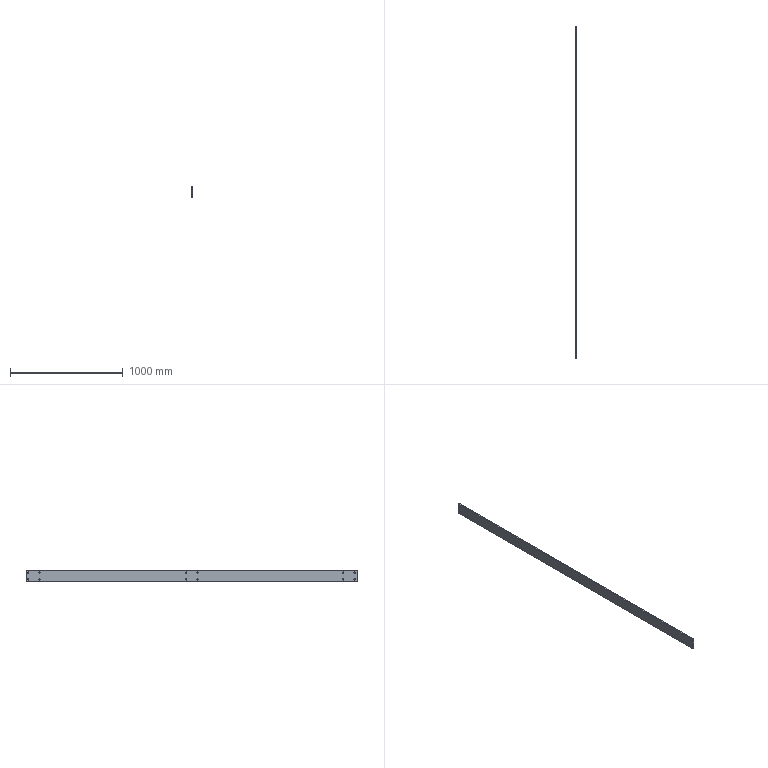Component | SolidWorks | Kick2-2 | 1 solid | 30 faces | box 10 x 2943.5 x 100 mm | volume 2932096 mm3 | cylinder 24 | plane 6 | commonest cylinder face diameters 11 x24 | material Plain Carbon Steel
STEP:
#1=COLOUR_RGB('',0.7922,0.8196,0.9333);
#2=FILL_AREA_STYLE_COLOUR('',#1);
#3=FILL_AREA_STYLE('',(#2));
#4=SURFACE_STYLE_FILL_AREA(#3);
#5=SURFACE_SIDE_STYLE('',(#4));
#6=SURFACE_STYLE_USAGE(.BOTH.,#5);
#7=PRESENTATION_STYLE_ASSIGNMENT((#6));
#8=CARTESIAN_POINT('',(-133.157,36.017,220.491));
#9=VERTEX_POINT('',#8);
#10=CARTESIAN_POINT('',(-133.157,36.017,220.924));
#11=VERTEX_POINT('',#10);
#12=CARTESIAN_POINT('',(-133.157,36.017,220.708));
#13=DIRECTION('',(-1.,0.,-0.));
#14=DIRECTION('',(0.,0.,-1.));
#15=AXIS2_PLACEMENT_3D('',#12,#13,#14);
#16=CIRCLE('',#15,0.2165);
#17=EDGE_CURVE('',#9,#11,#16,.T.);
#18=ORIENTED_EDGE('',*,*,#17,.T.);
#19=CARTESIAN_POINT('',(-132.764,36.017,220.924));
#20=VERTEX_POINT('',#19);
#21=CARTESIAN_POINT('',(-133.157,36.017,220.924));
#22=DIRECTION('',(1.,-0.,0.));
#23=VECTOR('',#22,39.37);
#24=LINE('',#21,#23);
#25=EDGE_CURVE('',#11,#20,#24,.T.);
#26=ORIENTED_EDGE('',*,*,#25,.T.);
#27=CARTESIAN_POINT('',(-132.764,36.017,220.491));
#28=VERTEX_POINT('',#27);
#29=CARTESIAN_POINT('',(-132.764,36.017,220.708));
#30=DIRECTION('',(1.,-0.,0.));
#31=DIRECTION('',(0.,0.,-1.));
#32=AXIS2_PLACEMENT_3D('',#29,#30,#31);
#33=CIRCLE('',#32,0.2165);
#34=EDGE_CURVE('',#20,#28,#33,.T.);
#35=ORIENTED_EDGE('',*,*,#34,.T.);
#36=CARTESIAN_POINT('',(-133.157,36.017,220.491));
#37=DIRECTION('',(1.,-0.,0.));
#38=VECTOR('',#37,39.37);
#39=LINE('',#36,#38);
#40=EDGE_CURVE('',#9,#28,#39,.T.);
#41=ORIENTED_EDGE('',*,*,#40,.F.);
#42=EDGE_LOOP('',(#18,#26,#35,#41));
#43=FACE_OUTER_BOUND('',#42,.T.);
#44=CARTESIAN_POINT('',(-133.157,36.017,220.708));
#45=DIRECTION('',(1.,-0.,0.));
#46=DIRECTION('',(0.,0.,-1.));
#47=AXIS2_PLACEMENT_3D('',#44,#45,#46);
#48=CYLINDRICAL_SURFACE('',#47,0.2165);
#49=ADVANCED_FACE('',(#43),#48,.F.);
#50=CARTESIAN_POINT('',(-133.157,32.08,220.491));
#51=VERTEX_POINT('',#50);
#52=CARTESIAN_POINT('',(-133.157,32.08,220.924));
#53=VERTEX_POINT('',#52);
#54=CARTESIAN_POINT('',(-133.157,32.08,220.708));
#55=DIRECTION('',(-1.,0.,-0.));
#56=DIRECTION('',(0.,0.,-1.));
#57=AXIS2_PLACEMENT_3D('',#54,#55,#56);
#58=CIRCLE('',#57,0.2165);
#59=EDGE_CURVE('',#51,#53,#58,.T.);
#60=ORIENTED_EDGE('',*,*,#59,.T.);
#61=CARTESIAN_POINT('',(-132.764,32.08,220.924));
#62=VERTEX_POINT('',#61);
#63=CARTESIAN_POINT('',(-133.157,32.08,220.924));
#64=DIRECTION('',(1.,-0.,0.));
#65=VECTOR('',#64,39.37);
#66=LINE('',#63,#65);
#67=EDGE_CURVE('',#53,#62,#66,.T.);
#68=ORIENTED_EDGE('',*,*,#67,.T.);
#69=CARTESIAN_POINT('',(-132.764,32.08,220.491));
#70=VERTEX_POINT('',#69);
#71=CARTESIAN_POINT('',(-132.764,32.08,220.708));
#72=DIRECTION('',(1.,-0.,0.));
#73=DIRECTION('',(0.,0.,-1.));
#74=AXIS2_PLACEMENT_3D('',#71,#72,#73);
#75=CIRCLE('',#74,0.2165);
#76=EDGE_CURVE('',#62,#70,#75,.T.);
#77=ORIENTED_EDGE('',*,*,#76,.T.);
#78=CARTESIAN_POINT('',(-133.157,32.08,220.491));
#79=DIRECTION('',(1.,-0.,0.));
#80=VECTOR('',#79,39.37);
#81=LINE('',#78,#80);
#82=EDGE_CURVE('',#51,#70,#81,.T.);
#83=ORIENTED_EDGE('',*,*,#82,.F.);
#84=EDGE_LOOP('',(#60,#68,#77,#83));
#85=FACE_OUTER_BOUND('',#84,.T.);
#86=CARTESIAN_POINT('',(-133.157,32.08,220.708));
#87=DIRECTION('',(1.,-0.,0.));
#88=DIRECTION('',(0.,0.,-1.));
#89=AXIS2_PLACEMENT_3D('',#86,#87,#88);
#90=CYLINDRICAL_SURFACE('',#89,0.2165);
#91=ADVANCED_FACE('',(#85),#90,.F.);
#92=CARTESIAN_POINT('',(-133.157,32.08,222.853));
#93=VERTEX_POINT('',#92);
#94=CARTESIAN_POINT('',(-133.157,32.08,223.286));
#95=VERTEX_POINT('',#94);
#96=CARTESIAN_POINT('',(-133.157,32.08,223.07));
#97=DIRECTION('',(-1.,0.,-0.));
#98=DIRECTION('',(0.,0.,-1.));
#99=AXIS2_PLACEMENT_3D('',#96,#97,#98);
#100=CIRCLE('',#99,0.2165);
#101=EDGE_CURVE('',#93,#95,#100,.T.);
#102=ORIENTED_EDGE('',*,*,#101,.T.);
#103=CARTESIAN_POINT('',(-132.764,32.08,223.286));
#104=VERTEX_POINT('',#103);
#105=CARTESIAN_POINT('',(-133.157,32.08,223.286));
#106=DIRECTION('',(1.,-0.,0.));
#107=VECTOR('',#106,39.37);
#108=LINE('',#105,#107);
#109=EDGE_CURVE('',#95,#104,#108,.T.);
#110=ORIENTED_EDGE('',*,*,#109,.T.);
#111=CARTESIAN_POINT('',(-132.764,32.08,222.853));
#112=VERTEX_POINT('',#111);
#113=CARTESIAN_POINT('',(-132.764,32.08,223.07));
#114=DIRECTION('',(1.,-0.,0.));
#115=DIRECTION('',(0.,0.,-1.));
#116=AXIS2_PLACEMENT_3D('',#113,#114,#115);
#117=CIRCLE('',#116,0.2165);
#118=EDGE_CURVE('',#104,#112,#117,.T.);
#119=ORIENTED_EDGE('',*,*,#118,.T.);
#120=CARTESIAN_POINT('',(-133.157,32.08,222.853));
#121=DIRECTION('',(1.,-0.,0.));
#122=VECTOR('',#121,39.37);
#123=LINE('',#120,#122);
#124=EDGE_CURVE('',#93,#112,#123,.T.);
#125=ORIENTED_EDGE('',*,*,#124,.F.);
#126=EDGE_LOOP('',(#102,#110,#119,#125));
#127=FACE_OUTER_BOUND('',#126,.T.);
#128=CARTESIAN_POINT('',(-133.157,32.08,223.07));
#129=DIRECTION('',(1.,-0.,0.));
#130=DIRECTION('',(0.,0.,-1.));
#131=AXIS2_PLACEMENT_3D('',#128,#129,#130);
#132=CYLINDRICAL_SURFACE('',#131,0.2165);
#133=ADVANCED_FACE('',(#127),#132,.F.);
#134=CARTESIAN_POINT('',(-133.157,-18.846,220.491));
#135=VERTEX_POINT('',#134);
#136=CARTESIAN_POINT('',(-133.157,-18.846,220.924));
#137=VERTEX_POINT('',#136);
#138=CARTESIAN_POINT('',(-133.157,-18.846,220.708));
#139=DIRECTION('',(-1.,0.,-0.));
#140=DIRECTION('',(0.,0.,-1.));
#141=AXIS2_PLACEMENT_3D('',#138,#139,#140);
#142=CIRCLE('',#141,0.2165);
#143=EDGE_CURVE('',#135,#137,#142,.T.);
#144=ORIENTED_EDGE('',*,*,#143,.T.);
#145=CARTESIAN_POINT('',(-132.764,-18.846,220.924));
#146=VERTEX_POINT('',#145);
#147=CARTESIAN_POINT('',(-133.157,-18.846,220.924));
#148=DIRECTION('',(1.,-0.,0.));
#149=VECTOR('',#148,39.37);
#150=LINE('',#147,#149);
#151=EDGE_CURVE('',#137,#146,#150,.T.);
#152=ORIENTED_EDGE('',*,*,#151,.T.);
#153=CARTESIAN_POINT('',(-132.764,-18.846,220.491));
#154=VERTEX_POINT('',#153);
#155=CARTESIAN_POINT('',(-132.764,-18.846,220.708));
#156=DIRECTION('',(1.,-0.,0.));
#157=DIRECTION('',(0.,0.,-1.));
#158=AXIS2_PLACEMENT_3D('',#155,#156,#157);
#159=CIRCLE('',#158,0.2165);
#160=EDGE_CURVE('',#146,#154,#159,.T.);
#161=ORIENTED_EDGE('',*,*,#160,.T.);
#162=CARTESIAN_POINT('',(-133.157,-18.846,220.491));
#163=DIRECTION('',(1.,-0.,0.));
#164=VECTOR('',#163,39.37);
#165=LINE('',#162,#164);
#166=EDGE_CURVE('',#135,#154,#165,.T.);
#167=ORIENTED_EDGE('',*,*,#166,.F.);
#168=EDGE_LOOP('',(#144,#152,#161,#167));
#169=FACE_OUTER_BOUND('',#168,.T.);
#170=CARTESIAN_POINT('',(-133.157,-18.846,220.708));
#171=DIRECTION('',(1.,-0.,0.));
#172=DIRECTION('',(0.,0.,-1.));
#173=AXIS2_PLACEMENT_3D('',#170,#171,#172);
#174=CYLINDRICAL_SURFACE('',#173,0.2165);
#175=ADVANCED_FACE('',(#169),#174,.F.);
#176=CARTESIAN_POINT('',(-133.157,91.135,222.853));
#177=VERTEX_POINT('',#176);
#178=CARTESIAN_POINT('',(-133.157,91.135,223.286));
#179=VERTEX_POINT('',#178);
#180=CARTESIAN_POINT('',(-133.157,91.135,223.07));
#181=DIRECTION('',(-1.,0.,-0.));
#182=DIRECTION('',(0.,0.,-1.));
#183=AXIS2_PLACEMENT_3D('',#180,#181,#182);
#184=CIRCLE('',#183,0.2165);
#185=EDGE_CURVE('',#177,#179,#184,.T.);
#186=ORIENTED_EDGE('',*,*,#185,.T.);
#187=CARTESIAN_POINT('',(-132.764,91.135,223.286));
#188=VERTEX_POINT('',#187);
#189=CARTESIAN_POINT('',(-133.157,91.135,223.286));
#190=DIRECTION('',(1.,-0.,0.));
#191=VECTOR('',#190,39.37);
#192=LINE('',#189,#191);
#193=EDGE_CURVE('',#179,#188,#192,.T.);
#194=ORIENTED_EDGE('',*,*,#193,.T.);
#195=CARTESIAN_POINT('',(-132.764,91.135,222.853));
#196=VERTEX_POINT('',#195);
#197=CARTESIAN_POINT('',(-132.764,91.135,223.07));
#198=DIRECTION('',(1.,-0.,0.));
#199=DIRECTION('',(0.,0.,-1.));
#200=AXIS2_PLACEMENT_3D('',#197,#198,#199);
#201=CIRCLE('',#200,0.2165);
#202=EDGE_CURVE('',#188,#196,#201,.T.);
#203=ORIENTED_EDGE('',*,*,#202,.T.);
#204=CARTESIAN_POINT('',(-133.157,91.135,222.853));
#205=DIRECTION('',(1.,-0.,0.));
#206=VECTOR('',#205,39.37);
#207=LINE('',#204,#206);
#208=EDGE_CURVE('',#177,#196,#207,.T.);
#209=ORIENTED_EDGE('',*,*,#208,.F.);
#210=EDGE_LOOP('',(#186,#194,#203,#209));
#211=FACE_OUTER_BOUND('',#210,.T.);
#212=CARTESIAN_POINT('',(-133.157,91.135,223.07));
#213=DIRECTION('',(1.,-0.,0.));
#214=DIRECTION('',(0.,0.,-1.));
#215=AXIS2_PLACEMENT_3D('',#212,#213,#214);
#216=CYLINDRICAL_SURFACE('',#215,0.2165);
#217=ADVANCED_FACE('',(#211),#216,.F.);
#218=CARTESIAN_POINT('',(-133.157,87.198,220.491));
#219=VERTEX_POINT('',#218);
#220=CARTESIAN_POINT('',(-133.157,87.198,220.924));
#221=VERTEX_POINT('',#220);
#222=CARTESIAN_POINT('',(-133.157,87.198,220.708));
#223=DIRECTION('',(-1.,0.,-0.));
#224=DIRECTION('',(0.,0.,-1.));
#225=AXIS2_PLACEMENT_3D('',#222,#223,#224);
#226=CIRCLE('',#225,0.2165);
#227=EDGE_CURVE('',#219,#221,#226,.T.);
#228=ORIENTED_EDGE('',*,*,#227,.T.);
#229=CARTESIAN_POINT('',(-132.764,87.198,220.924));
#230=VERTEX_POINT('',#229);
#231=CARTESIAN_POINT('',(-133.157,87.198,220.924));
#232=DIRECTION('',(1.,-0.,0.));
#233=VECTOR('',#232,39.37);
#234=LINE('',#231,#233);
#235=EDGE_CURVE('',#221,#230,#234,.T.);
#236=ORIENTED_EDGE('',*,*,#235,.T.);
#237=CARTESIAN_POINT('',(-132.764,87.198,220.491));
#238=VERTEX_POINT('',#237);
#239=CARTESIAN_POINT('',(-132.764,87.198,220.708));
#240=DIRECTION('',(1.,-0.,0.));
#241=DIRECTION('',(0.,0.,-1.));
#242=AXIS2_PLACEMENT_3D('',#239,#240,#241);
#243=CIRCLE('',#242,0.2165);
#244=EDGE_CURVE('',#230,#238,#243,.T.);
#245=ORIENTED_EDGE('',*,*,#244,.T.);
#246=CARTESIAN_POINT('',(-133.157,87.198,220.491));
#247=DIRECTION('',(1.,-0.,0.));
#248=VECTOR('',#247,39.37);
#249=LINE('',#246,#248);
#250=EDGE_CURVE('',#219,#238,#249,.T.);
#251=ORIENTED_EDGE('',*,*,#250,.F.);
#252=EDGE_LOOP('',(#228,#236,#245,#251));
#253=FACE_OUTER_BOUND('',#252,.T.);
#254=CARTESIAN_POINT('',(-133.157,87.198,220.708));
#255=DIRECTION('',(1.,-0.,0.));
#256=DIRECTION('',(0.,0.,-1.));
#257=AXIS2_PLACEMENT_3D('',#254,#255,#256);
#258=CYLINDRICAL_SURFACE('',#257,0.2165);
#259=ADVANCED_FACE('',(#253),#258,.F.);
#260=CARTESIAN_POINT('',(-133.157,87.198,222.853));
#261=VERTEX_POINT('',#260);
#262=CARTESIAN_POINT('',(-133.157,87.198,223.286));
#263=VERTEX_POINT('',#262);
#264=CARTESIAN_POINT('',(-133.157,87.198,223.07));
#265=DIRECTION('',(-1.,0.,-0.));
#266=DIRECTION('',(0.,0.,-1.));
#267=AXIS2_PLACEMENT_3D('',#264,#265,#266);
#268=CIRCLE('',#267,0.2165);
#269=EDGE_CURVE('',#261,#263,#268,.T.);
#270=ORIENTED_EDGE('',*,*,#269,.T.);
#271=CARTESIAN_POINT('',(-132.764,87.198,223.286));
#272=VERTEX_POINT('',#271);
#273=CARTESIAN_POINT('',(-133.157,87.198,223.286));
#274=DIRECTION('',(1.,-0.,0.));
#275=VECTOR('',#274,39.37);
#276=LINE('',#273,#275);
#277=EDGE_CURVE('',#263,#272,#276,.T.);
#278=ORIENTED_EDGE('',*,*,#277,.T.);
#279=CARTESIAN_POINT('',(-132.764,87.198,222.853));
#280=VERTEX_POINT('',#279);
#281=CARTESIAN_POINT('',(-132.764,87.198,223.07));
#282=DIRECTION('',(1.,-0.,0.));
#283=DIRECTION('',(0.,0.,-1.));
#284=AXIS2_PLACEMENT_3D('',#281,#282,#283);
#285=CIRCLE('',#284,0.2165);
#286=EDGE_CURVE('',#272,#280,#285,.T.);
#287=ORIENTED_EDGE('',*,*,#286,.T.);
#288=CARTESIAN_POINT('',(-133.157,87.198,222.853));
#289=DIRECTION('',(1.,-0.,0.));
#290=VECTOR('',#289,39.37);
#291=LINE('',#288,#290);
#292=EDGE_CURVE('',#261,#280,#291,.T.);
#293=ORIENTED_EDGE('',*,*,#292,.F.);
#294=EDGE_LOOP('',(#270,#278,#287,#293));
#295=FACE_OUTER_BOUND('',#294,.T.);
#296=CARTESIAN_POINT('',(-133.157,87.198,223.07));
#297=DIRECTION('',(1.,-0.,0.));
#298=DIRECTION('',(0.,0.,-1.));
#299=AXIS2_PLACEMENT_3D('',#296,#297,#298);
#300=CYLINDRICAL_SURFACE('',#299,0.2165);
#301=ADVANCED_FACE('',(#295),#300,.F.);
#302=CARTESIAN_POINT('',(-133.157,36.017,222.853));
#303=VERTEX_POINT('',#302);
#304=CARTESIAN_POINT('',(-133.157,36.017,223.286));
#305=VERTEX_POINT('',#304);
#306=CARTESIAN_POINT('',(-133.157,36.017,223.07));
#307=DIRECTION('',(-1.,0.,-0.));
#308=DIRECTION('',(0.,0.,-1.));
#309=AXIS2_PLACEMENT_3D('',#306,#307,#308);
#310=CIRCLE('',#309,0.2165);
#311=EDGE_CURVE('',#303,#305,#310,.T.);
#312=ORIENTED_EDGE('',*,*,#311,.T.);
#313=CARTESIAN_POINT('',(-132.764,36.017,223.286));
#314=VERTEX_POINT('',#313);
#315=CARTESIAN_POINT('',(-133.157,36.017,223.286));
#316=DIRECTION('',(1.,-0.,0.));
#317=VECTOR('',#316,39.37);
#318=LINE('',#315,#317);
#319=EDGE_CURVE('',#305,#314,#318,.T.);
#320=ORIENTED_EDGE('',*,*,#319,.T.);
#321=CARTESIAN_POINT('',(-132.764,36.017,222.853));
#322=VERTEX_POINT('',#321);
#323=CARTESIAN_POINT('',(-132.764,36.017,223.07));
#324=DIRECTION('',(1.,-0.,0.));
#325=DIRECTION('',(0.,0.,-1.));
#326=AXIS2_PLACEMENT_3D('',#323,#324,#325);
#327=CIRCLE('',#326,0.2165);
#328=EDGE_CURVE('',#314,#322,#327,.T.);
#329=ORIENTED_EDGE('',*,*,#328,.T.);
#330=CARTESIAN_POINT('',(-133.157,36.017,222.853));
#331=DIRECTION('',(1.,-0.,0.));
#332=VECTOR('',#331,39.37);
#333=LINE('',#330,#332);
#334=EDGE_CURVE('',#303,#322,#333,.T.);
#335=ORIENTED_EDGE('',*,*,#334,.F.);
#336=EDGE_LOOP('',(#312,#320,#329,#335));
#337=FACE_OUTER_BOUND('',#336,.T.);
#338=CARTESIAN_POINT('',(-133.157,36.017,223.07));
#339=DIRECTION('',(1.,-0.,0.));
#340=DIRECTION('',(0.,0.,-1.));
#341=AXIS2_PLACEMENT_3D('',#338,#339,#340);
#342=CYLINDRICAL_SURFACE('',#341,0.2165);
#343=ADVANCED_FACE('',(#337),#342,.F.);
#344=CARTESIAN_POINT('',(-133.157,-22.783,222.853));
#345=VERTEX_POINT('',#344);
#346=CARTESIAN_POINT('',(-133.157,-22.783,223.286));
#347=VERTEX_POINT('',#346);
#348=CARTESIAN_POINT('',(-133.157,-22.783,223.07));
#349=DIRECTION('',(-1.,0.,-0.));
#350=DIRECTION('',(0.,0.,-1.));
#351=AXIS2_PLACEMENT_3D('',#348,#349,#350);
#352=CIRCLE('',#351,0.2165);
#353=EDGE_CURVE('',#345,#347,#352,.T.);
#354=ORIENTED_EDGE('',*,*,#353,.T.);
#355=CARTESIAN_POINT('',(-132.764,-22.783,223.286));
#356=VERTEX_POINT('',#355);
#357=CARTESIAN_POINT('',(-133.157,-22.783,223.286));
#358=DIRECTION('',(1.,-0.,0.));
#359=VECTOR('',#358,39.37);
#360=LINE('',#357,#359);
#361=EDGE_CURVE('',#347,#356,#360,.T.);
#362=ORIENTED_EDGE('',*,*,#361,.T.);
#363=CARTESIAN_POINT('',(-132.764,-22.783,222.853));
#364=VERTEX_POINT('',#363);
#365=CARTESIAN_POINT('',(-132.764,-22.783,223.07));
#366=DIRECTION('',(1.,-0.,0.));
#367=DIRECTION('',(0.,0.,-1.));
#368=AXIS2_PLACEMENT_3D('',#365,#366,#367);
#369=CIRCLE('',#368,0.2165);
#370=EDGE_CURVE('',#356,#364,#369,.T.);
#371=ORIENTED_EDGE('',*,*,#370,.T.);
#372=CARTESIAN_POINT('',(-133.157,-22.783,222.853));
#373=DIRECTION('',(1.,-0.,0.));
#374=VECTOR('',#373,39.37);
#375=LINE('',#372,#374);
#376=EDGE_CURVE('',#345,#364,#375,.T.);
#377=ORIENTED_EDGE('',*,*,#376,.F.);
#378=EDGE_LOOP('',(#354,#362,#371,#377));
#379=FACE_OUTER_BOUND('',#378,.T.);
#380=CARTESIAN_POINT('',(-133.157,-22.783,223.07));
#381=DIRECTION('',(1.,-0.,0.));
#382=DIRECTION('',(0.,0.,-1.));
#383=AXIS2_PLACEMENT_3D('',#380,#381,#382);
#384=CYLINDRICAL_SURFACE('',#383,0.2165);
#385=ADVANCED_FACE('',(#379),#384,.F.);
#386=CARTESIAN_POINT('',(-133.157,-22.783,220.491));
#387=VERTEX_POINT('',#386);
#388=CARTESIAN_POINT('',(-133.157,-22.783,220.924));
#389=VERTEX_POINT('',#388);
#390=CARTESIAN_POINT('',(-133.157,-22.783,220.708));
#391=DIRECTION('',(-1.,0.,-0.));
#392=DIRECTION('',(0.,0.,-1.));
#393=AXIS2_PLACEMENT_3D('',#390,#391,#392);
#394=CIRCLE('',#393,0.2165);
#395=EDGE_CURVE('',#387,#389,#394,.T.);
#396=ORIENTED_EDGE('',*,*,#395,.T.);
#397=CARTESIAN_POINT('',(-132.764,-22.783,220.924));
#398=VERTEX_POINT('',#397);
#399=CARTESIAN_POINT('',(-133.157,-22.783,220.924));
#400=DIRECTION('',(1.,-0.,0.));
#401=VECTOR('',#400,39.37);
#402=LINE('',#399,#401);
#403=EDGE_CURVE('',#389,#398,#402,.T.);
#404=ORIENTED_EDGE('',*,*,#403,.T.);
#405=CARTESIAN_POINT('',(-132.764,-22.783,220.491));
#406=VERTEX_POINT('',#405);
#407=CARTESIAN_POINT('',(-132.764,-22.783,220.708));
#408=DIRECTION('',(1.,-0.,0.));
#409=DIRECTION('',(0.,0.,-1.));
#410=AXIS2_PLACEMENT_3D('',#407,#408,#409);
#411=CIRCLE('',#410,0.2165);
#412=EDGE_CURVE('',#398,#406,#411,.T.);
#413=ORIENTED_EDGE('',*,*,#412,.T.);
#414=CARTESIAN_POINT('',(-133.157,-22.783,220.491));
#415=DIRECTION('',(1.,-0.,0.));
#416=VECTOR('',#415,39.37);
#417=LINE('',#414,#416);
#418=EDGE_CURVE('',#387,#406,#417,.T.);
#419=ORIENTED_EDGE('',*,*,#418,.F.);
#420=EDGE_LOOP('',(#396,#404,#413,#419));
#421=FACE_OUTER_BOUND('',#420,.T.);
#422=CARTESIAN_POINT('',(-133.157,-22.783,220.708));
#423=DIRECTION('',(1.,-0.,0.));
#424=DIRECTION('',(0.,0.,-1.));
#425=AXIS2_PLACEMENT_3D('',#422,#423,#424);
#426=CYLINDRICAL_SURFACE('',#425,0.2165);
#427=ADVANCED_FACE('',(#421),#426,.F.);
#428=CARTESIAN_POINT('',(-133.157,-18.846,222.853));
#429=VERTEX_POINT('',#428);
#430=CARTESIAN_POINT('',(-133.157,-18.846,223.286));
#431=VERTEX_POINT('',#430);
#432=CARTESIAN_POINT('',(-133.157,-18.846,223.07));
#433=DIRECTION('',(-1.,0.,-0.));
#434=DIRECTION('',(0.,0.,-1.));
#435=AXIS2_PLACEMENT_3D('',#432,#433,#434);
#436=CIRCLE('',#435,0.2165);
#437=EDGE_CURVE('',#429,#431,#436,.T.);
#438=ORIENTED_EDGE('',*,*,#437,.T.);
#439=CARTESIAN_POINT('',(-132.764,-18.846,223.286));
#440=VERTEX_POINT('',#439);
#441=CARTESIAN_POINT('',(-133.157,-18.846,223.286));
#442=DIRECTION('',(1.,-0.,0.));
#443=VECTOR('',#442,39.37);
#444=LINE('',#441,#443);
#445=EDGE_CURVE('',#431,#440,#444,.T.);
#446=ORIENTED_EDGE('',*,*,#445,.T.);
#447=CARTESIAN_POINT('',(-132.764,-18.846,222.853));
#448=VERTEX_POINT('',#447);
#449=CARTESIAN_POINT('',(-132.764,-18.846,223.07));
#450=DIRECTION('',(1.,-0.,0.));
#451=DIRECTION('',(0.,0.,-1.));
#452=AXIS2_PLACEMENT_3D('',#449,#450,#451);
#453=CIRCLE('',#452,0.2165);
#454=EDGE_CURVE('',#440,#448,#453,.T.);
#455=ORIENTED_EDGE('',*,*,#454,.T.);
#456=CARTESIAN_POINT('',(-133.157,-18.846,222.853));
#457=DIRECTION('',(1.,-0.,0.));
#458=VECTOR('',#457,39.37);
#459=LINE('',#456,#458);
#460=EDGE_CURVE('',#429,#448,#459,.T.);
#461=ORIENTED_EDGE('',*,*,#460,.F.);
#462=EDGE_LOOP('',(#438,#446,#455,#461));
#463=FACE_OUTER_BOUND('',#462,.T.);
#464=CARTESIAN_POINT('',(-133.157,-18.846,223.07));
#465=DIRECTION('',(1.,-0.,0.));
#466=DIRECTION('',(0.,0.,-1.));
#467=AXIS2_PLACEMENT_3D('',#464,#465,#466);
#468=CYLINDRICAL_SURFACE('',#467,0.2165);
#469=ADVANCED_FACE('',(#463),#468,.F.);
#470=CARTESIAN_POINT('',(-133.157,91.135,220.491));
#471=VERTEX_POINT('',#470);
#472=CARTESIAN_POINT('',(-133.157,91.135,220.924));
#473=VERTEX_POINT('',#472);
#474=CARTESIAN_POINT('',(-133.157,91.135,220.708));
#475=DIRECTION('',(-1.,0.,-0.));
#476=DIRECTION('',(0.,0.,-1.));
#477=AXIS2_PLACEMENT_3D('',#474,#475,#476);
#478=CIRCLE('',#477,0.2165);
#479=EDGE_CURVE('',#471,#473,#478,.T.);
#480=ORIENTED_EDGE('',*,*,#479,.T.);
#481=CARTESIAN_POINT('',(-132.764,91.135,220.924));
#482=VERTEX_POINT('',#481);
#483=CARTESIAN_POINT('',(-133.157,91.135,220.924));
#484=DIRECTION('',(1.,-0.,0.));
#485=VECTOR('',#484,39.37);
#486=LINE('',#483,#485);
#487=EDGE_CURVE('',#473,#482,#486,.T.);
#488=ORIENTED_EDGE('',*,*,#487,.T.);
#489=CARTESIAN_POINT('',(-132.764,91.135,220.491));
#490=VERTEX_POINT('',#489);
#491=CARTESIAN_POINT('',(-132.764,91.135,220.708));
#492=DIRECTION('',(1.,-0.,0.));
#493=DIRECTION('',(0.,0.,-1.));
#494=AXIS2_PLACEMENT_3D('',#491,#492,#493);
#495=CIRCLE('',#494,0.2165);
#496=EDGE_CURVE('',#482,#490,#495,.T.);
#497=ORIENTED_EDGE('',*,*,#496,.T.);
#498=CARTESIAN_POINT('',(-133.157,91.135,220.491));
#499=DIRECTION('',(1.,-0.,0.));
#500=VECTOR('',#499,39.37);
#501=LINE('',#498,#500);
#502=EDGE_CURVE('',#471,#490,#501,.T.);
#503=ORIENTED_EDGE('',*,*,#502,.F.);
#504=EDGE_LOOP('',(#480,#488,#497,#503));
#505=FACE_OUTER_BOUND('',#504,.T.);
#506=CARTESIAN_POINT('',(-133.157,91.135,220.708));
#507=DIRECTION('',(1.,-0.,0.));
#508=DIRECTION('',(0.,0.,-1.));
#509=AXIS2_PLACEMENT_3D('',#506,#507,#508);
#510=CYLINDRICAL_SURFACE('',#509,0.2165);
#511=ADVANCED_FACE('',(#505),#510,.F.);
#512=CARTESIAN_POINT('',(-132.764,-23.964,223.857));
#513=VERTEX_POINT('',#512);
#514=CARTESIAN_POINT('',(-132.764,-23.964,219.92));
#515=VERTEX_POINT('',#514);
#516=CARTESIAN_POINT('',(-132.764,-23.964,223.857));
#517=DIRECTION('',(0.,0.,-1.));
#518=VECTOR('',#517,39.37);
#519=LINE('',#516,#518);
#520=EDGE_CURVE('',#513,#515,#519,.T.);
#521=ORIENTED_EDGE('',*,*,#520,.F.);
#522=CARTESIAN_POINT('',(-133.157,-23.964,223.857));
#523=VERTEX_POINT('',#522);
#524=CARTESIAN_POINT('',(-133.157,-23.964,223.857));
#525=DIRECTION('',(1.,-0.,0.));
#526=VECTOR('',#525,39.37);
#527=LINE('',#524,#526);
#528=EDGE_CURVE('',#523,#513,#527,.T.);
#529=ORIENTED_EDGE('',*,*,#528,.F.);
#530=CARTESIAN_POINT('',(-133.157,-23.964,219.92));
#531=VERTEX_POINT('',#530);
#532=CARTESIAN_POINT('',(-133.157,-23.964,223.857));
#533=DIRECTION('',(0.,0.,-1.));
#534=VECTOR('',#533,39.37);
#535=LINE('',#532,#534);
#536=EDGE_CURVE('',#523,#531,#535,.T.);
#537=ORIENTED_EDGE('',*,*,#536,.T.);
#538=CARTESIAN_POINT('',(-133.157,-23.964,219.92));
#539=DIRECTION('',(1.,-0.,0.));
#540=VECTOR('',#539,39.37);
#541=LINE('',#538,#540);
#542=EDGE_CURVE('',#531,#515,#541,.T.);
#543=ORIENTED_EDGE('',*,*,#542,.T.);
#544=EDGE_LOOP('',(#521,#529,#537,#543));
#545=FACE_OUTER_BOUND('',#544,.T.);
#546=CARTESIAN_POINT('',(-133.157,-23.964,223.857));
#547=DIRECTION('',(-0.,-1.,-0.));
#548=DIRECTION('',(0.,0.,-1.));
#549=AXIS2_PLACEMENT_3D('',#546,#547,#548);
#550=PLANE('',#549);
#551=ADVANCED_FACE('',(#545),#550,.T.);
#552=CARTESIAN_POINT('',(-132.764,91.922,223.857));
#553=VERTEX_POINT('',#552);
#554=CARTESIAN_POINT('',(-133.157,91.922,223.857));
#555=VERTEX_POINT('',#554);
#556=CARTESIAN_POINT('',(-132.764,91.922,223.857));
#557=DIRECTION('',(-1.,0.,-0.));
#558=VECTOR('',#557,39.37);
#559=LINE('',#556,#558);
#560=EDGE_CURVE('',#553,#555,#559,.T.);
#561=ORIENTED_EDGE('',*,*,#560,.T.);
#562=CARTESIAN_POINT('',(-133.157,-23.964,223.857));
#563=DIRECTION('',(-0.,-1.,-0.));
#564=VECTOR('',#563,39.37);
#565=LINE('',#562,#564);
#566=EDGE_CURVE('',#555,#523,#565,.T.);
#567=ORIENTED_EDGE('',*,*,#566,.T.);
#568=ORIENTED_EDGE('',*,*,#528,.T.);
#569=CARTESIAN_POINT('',(-132.764,-23.964,223.857));
#570=DIRECTION('',(-0.,-1.,-0.));
#571=VECTOR('',#570,39.37);
#572=LINE('',#569,#571);
#573=EDGE_CURVE('',#553,#513,#572,.T.);
#574=ORIENTED_EDGE('',*,*,#573,.F.);
#575=EDGE_LOOP('',(#561,#567,#568,#574));
#576=FACE_OUTER_BOUND('',#575,.T.);
#577=CARTESIAN_POINT('',(-133.157,-23.964,223.857));
#578=DIRECTION('',(-0.,-0.,1.));
#579=DIRECTION('',(-0.,-1.,-0.));
#580=AXIS2_PLACEMENT_3D('',#577,#578,#579);
#581=PLANE('',#580);
#582=ADVANCED_FACE('',(#576),#581,.T.);
#583=CARTESIAN_POINT('',(-132.764,91.922,219.92));
#584=VERTEX_POINT('',#583);
#585=CARTESIAN_POINT('',(-133.157,91.922,219.92));
#586=VERTEX_POINT('',#585);
#587=CARTESIAN_POINT('',(-132.764,91.922,219.92));
#588=DIRECTION('',(-1.,0.,-0.));
#589=VECTOR('',#588,39.37);
#590=LINE('',#587,#589);
#591=EDGE_CURVE('',#584,#586,#590,.T.);
#592=ORIENTED_EDGE('',*,*,#591,.F.);
#593=CARTESIAN_POINT('',(-132.764,-23.964,219.92));
#594=DIRECTION('',(0.,1.,-0.));
#595=VECTOR('',#594,39.37);
#596=LINE('',#593,#595);
#597=EDGE_CURVE('',#515,#584,#596,.T.);
#598=ORIENTED_EDGE('',*,*,#597,.F.);
#599=ORIENTED_EDGE('',*,*,#542,.F.);
#600=CARTESIAN_POINT('',(-133.157,-23.964,219.92));
#601=DIRECTION('',(0.,1.,-0.));
#602=VECTOR('',#601,39.37);
#603=LINE('',#600,#602);
#604=EDGE_CURVE('',#531,#586,#603,.T.);
#605=ORIENTED_EDGE('',*,*,#604,.T.);
#606=EDGE_LOOP('',(#592,#598,#599,#605));
#607=FACE_OUTER_BOUND('',#606,.T.);
#608=CARTESIAN_POINT('',(-133.157,-23.964,219.92));
#609=DIRECTION('',(0.,-0.,-1.));
#610=DIRECTION('',(0.,1.,-0.));
#611=AXIS2_PLACEMENT_3D('',#608,#609,#610);
#612=PLANE('',#611);
#613=ADVANCED_FACE('',(#607),#612,.T.);
#614=ORIENTED_EDGE('',*,*,#17,.F.);
#615=CARTESIAN_POINT('',(-133.157,36.017,220.708));
#616=DIRECTION('',(-1.,0.,-0.));
#617=DIRECTION('',(0.,0.,-1.));
#618=AXIS2_PLACEMENT_3D('',#615,#616,#617);
#619=CIRCLE('',#618,0.2165);
#620=EDGE_CURVE('',#11,#9,#619,.T.);
#621=ORIENTED_EDGE('',*,*,#620,.F.);
#622=EDGE_LOOP('',(#614,#621));
#623=FACE_BOUND('',#622,.T.);
#624=ORIENTED_EDGE('',*,*,#59,.F.);
#625=CARTESIAN_POINT('',(-133.157,32.08,220.708));
#626=DIRECTION('',(-1.,0.,-0.));
#627=DIRECTION('',(0.,0.,-1.));
#628=AXIS2_PLACEMENT_3D('',#625,#626,#627);
#629=CIRCLE('',#628,0.2165);
#630=EDGE_CURVE('',#53,#51,#629,.T.);
#631=ORIENTED_EDGE('',*,*,#630,.F.);
#632=EDGE_LOOP('',(#624,#631));
#633=FACE_BOUND('',#632,.T.);
#634=ORIENTED_EDGE('',*,*,#101,.F.);
#635=CARTESIAN_POINT('',(-133.157,32.08,223.07));
#636=DIRECTION('',(-1.,0.,-0.));
#637=DIRECTION('',(0.,0.,-1.));
#638=AXIS2_PLACEMENT_3D('',#635,#636,#637);
#639=CIRCLE('',#638,0.2165);
#640=EDGE_CURVE('',#95,#93,#639,.T.);
#641=ORIENTED_EDGE('',*,*,#640,.F.);
#642=EDGE_LOOP('',(#634,#641));
#643=FACE_BOUND('',#642,.T.);
#644=ORIENTED_EDGE('',*,*,#143,.F.);
#645=CARTESIAN_POINT('',(-133.157,-18.846,220.708));
#646=DIRECTION('',(-1.,0.,-0.));
#647=DIRECTION('',(0.,0.,-1.));
#648=AXIS2_PLACEMENT_3D('',#645,#646,#647);
#649=CIRCLE('',#648,0.2165);
#650=EDGE_CURVE('',#137,#135,#649,.T.);
#651=ORIENTED_EDGE('',*,*,#650,.F.);
#652=EDGE_LOOP('',(#644,#651));
#653=FACE_BOUND('',#652,.T.);
#654=ORIENTED_EDGE('',*,*,#185,.F.);
#655=CARTESIAN_POINT('',(-133.157,91.135,223.07));
#656=DIRECTION('',(-1.,0.,-0.));
#657=DIRECTION('',(0.,0.,-1.));
#658=AXIS2_PLACEMENT_3D('',#655,#656,#657);
#659=CIRCLE('',#658,0.2165);
#660=EDGE_CURVE('',#179,#177,#659,.T.);
#661=ORIENTED_EDGE('',*,*,#660,.F.);
#662=EDGE_LOOP('',(#654,#661));
#663=FACE_BOUND('',#662,.T.);
#664=ORIENTED_EDGE('',*,*,#227,.F.);
#665=CARTESIAN_POINT('',(-133.157,87.198,220.708));
#666=DIRECTION('',(-1.,0.,-0.));
#667=DIRECTION('',(0.,0.,-1.));
#668=AXIS2_PLACEMENT_3D('',#665,#666,#667);
#669=CIRCLE('',#668,0.2165);
#670=EDGE_CURVE('',#221,#219,#669,.T.);
#671=ORIENTED_EDGE('',*,*,#670,.F.);
#672=EDGE_LOOP('',(#664,#671));
#673=FACE_BOUND('',#672,.T.);
#674=ORIENTED_EDGE('',*,*,#269,.F.);
#675=CARTESIAN_POINT('',(-133.157,87.198,223.07));
#676=DIRECTION('',(-1.,0.,-0.));
#677=DIRECTION('',(0.,0.,-1.));
#678=AXIS2_PLACEMENT_3D('',#675,#676,#677);
#679=CIRCLE('',#678,0.2165);
#680=EDGE_CURVE('',#263,#261,#679,.T.);
#681=ORIENTED_EDGE('',*,*,#680,.F.);
#682=EDGE_LOOP('',(#674,#681));
#683=FACE_BOUND('',#682,.T.);
#684=ORIENTED_EDGE('',*,*,#311,.F.);
#685=CARTESIAN_POINT('',(-133.157,36.017,223.07));
#686=DIRECTION('',(-1.,0.,-0.));
#687=DIRECTION('',(0.,0.,-1.));
#688=AXIS2_PLACEMENT_3D('',#685,#686,#687);
#689=CIRCLE('',#688,0.2165);
#690=EDGE_CURVE('',#305,#303,#689,.T.);
#691=ORIENTED_EDGE('',*,*,#690,.F.);
#692=EDGE_LOOP('',(#684,#691));
#693=FACE_BOUND('',#692,.T.);
#694=ORIENTED_EDGE('',*,*,#353,.F.);
#695=CARTESIAN_POINT('',(-133.157,-22.783,223.07));
#696=DIRECTION('',(-1.,0.,-0.));
#697=DIRECTION('',(0.,0.,-1.));
#698=AXIS2_PLACEMENT_3D('',#695,#696,#697);
#699=CIRCLE('',#698,0.2165);
#700=EDGE_CURVE('',#347,#345,#699,.T.);
#701=ORIENTED_EDGE('',*,*,#700,.F.);
#702=EDGE_LOOP('',(#694,#701));
#703=FACE_BOUND('',#702,.T.);
#704=ORIENTED_EDGE('',*,*,#395,.F.);
#705=CARTESIAN_POINT('',(-133.157,-22.783,220.708));
#706=DIRECTION('',(-1.,0.,-0.));
#707=DIRECTION('',(0.,0.,-1.));
#708=AXIS2_PLACEMENT_3D('',#705,#706,#707);
#709=CIRCLE('',#708,0.2165);
#710=EDGE_CURVE('',#389,#387,#709,.T.);
#711=ORIENTED_EDGE('',*,*,#710,.F.);
#712=EDGE_LOOP('',(#704,#711));
#713=FACE_BOUND('',#712,.T.);
#714=ORIENTED_EDGE('',*,*,#437,.F.);
#715=CARTESIAN_POINT('',(-133.157,-18.846,223.07));
#716=DIRECTION('',(-1.,0.,-0.));
#717=DIRECTION('',(0.,0.,-1.));
#718=AXIS2_PLACEMENT_3D('',#715,#716,#717);
#719=CIRCLE('',#718,0.2165);
#720=EDGE_CURVE('',#431,#429,#719,.T.);
#721=ORIENTED_EDGE('',*,*,#720,.F.);
#722=EDGE_LOOP('',(#714,#721));
#723=FACE_BOUND('',#722,.T.);
#724=ORIENTED_EDGE('',*,*,#479,.F.);
#725=CARTESIAN_POINT('',(-133.157,91.135,220.708));
#726=DIRECTION('',(-1.,0.,-0.));
#727=DIRECTION('',(0.,0.,-1.));
#728=AXIS2_PLACEMENT_3D('',#725,#726,#727);
#729=CIRCLE('',#728,0.2165);
#730=EDGE_CURVE('',#473,#471,#729,.T.);
#731=ORIENTED_EDGE('',*,*,#730,.F.);
#732=EDGE_LOOP('',(#724,#731));
#733=FACE_BOUND('',#732,.T.);
#734=ORIENTED_EDGE('',*,*,#566,.F.);
#735=CARTESIAN_POINT('',(-133.157,91.922,219.92));
#736=DIRECTION('',(-0.,-0.,1.));
#737=VECTOR('',#736,39.37);
#738=LINE('',#735,#737);
#739=EDGE_CURVE('',#586,#555,#738,.T.);
#740=ORIENTED_EDGE('',*,*,#739,.F.);
#741=ORIENTED_EDGE('',*,*,#604,.F.);
#742=ORIENTED_EDGE('',*,*,#536,.F.);
#743=EDGE_LOOP('',(#734,#740,#741,#742));
#744=FACE_OUTER_BOUND('',#743,.T.);
#745=CARTESIAN_POINT('',(-133.157,-23.964,223.857));
#746=DIRECTION('',(1.,-0.,0.));
#747=DIRECTION('',(0.,0.,-1.));
#748=AXIS2_PLACEMENT_3D('',#745,#746,#747);
#749=PLANE('',#748);
#750=ADVANCED_FACE('',(#623,#633,#643,#653,#663,#673,#683,#693,#703,#713,#723,#733,#744),#749,.F.);
#751=CARTESIAN_POINT('',(-132.764,36.017,220.708));
#752=DIRECTION('',(1.,-0.,0.));
#753=DIRECTION('',(0.,0.,-1.));
#754=AXIS2_PLACEMENT_3D('',#751,#752,#753);
#755=CIRCLE('',#754,0.2165);
#756=EDGE_CURVE('',#28,#20,#755,.T.);
#757=ORIENTED_EDGE('',*,*,#756,.F.);
#758=ORIENTED_EDGE('',*,*,#34,.F.);
#759=EDGE_LOOP('',(#757,#758));
#760=FACE_BOUND('',#759,.T.);
#761=CARTESIAN_POINT('',(-132.764,32.08,220.708));
#762=DIRECTION('',(1.,-0.,0.));
#763=DIRECTION('',(0.,0.,-1.));
#764=AXIS2_PLACEMENT_3D('',#761,#762,#763);
#765=CIRCLE('',#764,0.2165);
#766=EDGE_CURVE('',#70,#62,#765,.T.);
#767=ORIENTED_EDGE('',*,*,#766,.F.);
#768=ORIENTED_EDGE('',*,*,#76,.F.);
#769=EDGE_LOOP('',(#767,#768));
#770=FACE_BOUND('',#769,.T.);
#771=CARTESIAN_POINT('',(-132.764,32.08,223.07));
#772=DIRECTION('',(1.,-0.,0.));
#773=DIRECTION('',(0.,0.,-1.));
#774=AXIS2_PLACEMENT_3D('',#771,#772,#773);
#775=CIRCLE('',#774,0.2165);
#776=EDGE_CURVE('',#112,#104,#775,.T.);
#777=ORIENTED_EDGE('',*,*,#776,.F.);
#778=ORIENTED_EDGE('',*,*,#118,.F.);
#779=EDGE_LOOP('',(#777,#778));
#780=FACE_BOUND('',#779,.T.);
#781=CARTESIAN_POINT('',(-132.764,-18.846,220.708));
#782=DIRECTION('',(1.,-0.,0.));
#783=DIRECTION('',(0.,0.,-1.));
#784=AXIS2_PLACEMENT_3D('',#781,#782,#783);
#785=CIRCLE('',#784,0.2165);
#786=EDGE_CURVE('',#154,#146,#785,.T.);
#787=ORIENTED_EDGE('',*,*,#786,.F.);
#788=ORIENTED_EDGE('',*,*,#160,.F.);
#789=EDGE_LOOP('',(#787,#788));
#790=FACE_BOUND('',#789,.T.);
#791=CARTESIAN_POINT('',(-132.764,91.135,223.07));
#792=DIRECTION('',(1.,-0.,0.));
#793=DIRECTION('',(0.,0.,-1.));
#794=AXIS2_PLACEMENT_3D('',#791,#792,#793);
#795=CIRCLE('',#794,0.2165);
#796=EDGE_CURVE('',#196,#188,#795,.T.);
#797=ORIENTED_EDGE('',*,*,#796,.F.);
#798=ORIENTED_EDGE('',*,*,#202,.F.);
#799=EDGE_LOOP('',(#797,#798));
#800=FACE_BOUND('',#799,.T.);
#801=CARTESIAN_POINT('',(-132.764,87.198,220.708));
#802=DIRECTION('',(1.,-0.,0.));
#803=DIRECTION('',(0.,0.,-1.));
#804=AXIS2_PLACEMENT_3D('',#801,#802,#803);
#805=CIRCLE('',#804,0.2165);
#806=EDGE_CURVE('',#238,#230,#805,.T.);
#807=ORIENTED_EDGE('',*,*,#806,.F.);
#808=ORIENTED_EDGE('',*,*,#244,.F.);
#809=EDGE_LOOP('',(#807,#808));
#810=FACE_BOUND('',#809,.T.);
#811=CARTESIAN_POINT('',(-132.764,87.198,223.07));
#812=DIRECTION('',(1.,-0.,0.));
#813=DIRECTION('',(0.,0.,-1.));
#814=AXIS2_PLACEMENT_3D('',#811,#812,#813);
#815=CIRCLE('',#814,0.2165);
#816=EDGE_CURVE('',#280,#272,#815,.T.);
#817=ORIENTED_EDGE('',*,*,#816,.F.);
#818=ORIENTED_EDGE('',*,*,#286,.F.);
#819=EDGE_LOOP('',(#817,#818));
#820=FACE_BOUND('',#819,.T.);
#821=CARTESIAN_POINT('',(-132.764,36.017,223.07));
#822=DIRECTION('',(1.,-0.,0.));
#823=DIRECTION('',(0.,0.,-1.));
#824=AXIS2_PLACEMENT_3D('',#821,#822,#823);
#825=CIRCLE('',#824,0.2165);
#826=EDGE_CURVE('',#322,#314,#825,.T.);
#827=ORIENTED_EDGE('',*,*,#826,.F.);
#828=ORIENTED_EDGE('',*,*,#328,.F.);
#829=EDGE_LOOP('',(#827,#828));
#830=FACE_BOUND('',#829,.T.);
#831=CARTESIAN_POINT('',(-132.764,-22.783,223.07));
#832=DIRECTION('',(1.,-0.,0.));
#833=DIRECTION('',(0.,0.,-1.));
#834=AXIS2_PLACEMENT_3D('',#831,#832,#833);
#835=CIRCLE('',#834,0.2165);
#836=EDGE_CURVE('',#364,#356,#835,.T.);
#837=ORIENTED_EDGE('',*,*,#836,.F.);
#838=ORIENTED_EDGE('',*,*,#370,.F.);
#839=EDGE_LOOP('',(#837,#838));
#840=FACE_BOUND('',#839,.T.);
#841=CARTESIAN_POINT('',(-132.764,-22.783,220.708));
#842=DIRECTION('',(1.,-0.,0.));
#843=DIRECTION('',(0.,0.,-1.));
#844=AXIS2_PLACEMENT_3D('',#841,#842,#843);
#845=CIRCLE('',#844,0.2165);
#846=EDGE_CURVE('',#406,#398,#845,.T.);
#847=ORIENTED_EDGE('',*,*,#846,.F.);
#848=ORIENTED_EDGE('',*,*,#412,.F.);
#849=EDGE_LOOP('',(#847,#848));
#850=FACE_BOUND('',#849,.T.);
#851=CARTESIAN_POINT('',(-132.764,-18.846,223.07));
#852=DIRECTION('',(1.,-0.,0.));
#853=DIRECTION('',(0.,0.,-1.));
#854=AXIS2_PLACEMENT_3D('',#851,#852,#853);
#855=CIRCLE('',#854,0.2165);
#856=EDGE_CURVE('',#448,#440,#855,.T.);
#857=ORIENTED_EDGE('',*,*,#856,.F.);
#858=ORIENTED_EDGE('',*,*,#454,.F.);
#859=EDGE_LOOP('',(#857,#858));
#860=FACE_BOUND('',#859,.T.);
#861=CARTESIAN_POINT('',(-132.764,91.135,220.708));
#862=DIRECTION('',(1.,-0.,0.));
#863=DIRECTION('',(0.,0.,-1.));
#864=AXIS2_PLACEMENT_3D('',#861,#862,#863);
#865=CIRCLE('',#864,0.2165);
#866=EDGE_CURVE('',#490,#482,#865,.T.);
#867=ORIENTED_EDGE('',*,*,#866,.F.);
#868=ORIENTED_EDGE('',*,*,#496,.F.);
#869=EDGE_LOOP('',(#867,#868));
#870=FACE_BOUND('',#869,.T.);
#871=CARTESIAN_POINT('',(-132.764,91.922,219.92));
#872=DIRECTION('',(-0.,-0.,1.));
#873=VECTOR('',#872,39.37);
#874=LINE('',#871,#873);
#875=EDGE_CURVE('',#584,#553,#874,.T.);
#876=ORIENTED_EDGE('',*,*,#875,.T.);
#877=ORIENTED_EDGE('',*,*,#573,.T.);
#878=ORIENTED_EDGE('',*,*,#520,.T.);
#879=ORIENTED_EDGE('',*,*,#597,.T.);
#880=EDGE_LOOP('',(#876,#877,#878,#879));
#881=FACE_OUTER_BOUND('',#880,.T.);
#882=CARTESIAN_POINT('',(-132.764,-23.964,223.857));
#883=DIRECTION('',(1.,-0.,0.));
#884=DIRECTION('',(0.,0.,-1.));
#885=AXIS2_PLACEMENT_3D('',#882,#883,#884);
#886=PLANE('',#885);
#887=ADVANCED_FACE('',(#760,#770,#780,#790,#800,#810,#820,#830,#840,#850,#860,#870,#881),#886,.T.);
#888=ORIENTED_EDGE('',*,*,#591,.T.);
#889=ORIENTED_EDGE('',*,*,#739,.T.);
#890=ORIENTED_EDGE('',*,*,#560,.F.);
#891=ORIENTED_EDGE('',*,*,#875,.F.);
#892=EDGE_LOOP('',(#888,#889,#890,#891));
#893=FACE_OUTER_BOUND('',#892,.T.);
#894=CARTESIAN_POINT('',(-132.764,91.922,219.92));
#895=DIRECTION('',(-0.,-1.,-0.));
#896=DIRECTION('',(0.,0.,-1.));
#897=AXIS2_PLACEMENT_3D('',#894,#895,#896);
#898=PLANE('',#897);
#899=ADVANCED_FACE('',(#893),#898,.F.);
#900=ORIENTED_EDGE('',*,*,#487,.F.);
#901=ORIENTED_EDGE('',*,*,#730,.T.);
#902=ORIENTED_EDGE('',*,*,#502,.T.);
#903=ORIENTED_EDGE('',*,*,#866,.T.);
#904=EDGE_LOOP('',(#900,#901,#902,#903));
#905=FACE_OUTER_BOUND('',#904,.T.);
#906=CARTESIAN_POINT('',(-133.157,91.135,220.708));
#907=DIRECTION('',(1.,-0.,0.));
#908=DIRECTION('',(0.,0.,-1.));
#909=AXIS2_PLACEMENT_3D('',#906,#907,#908);
#910=CYLINDRICAL_SURFACE('',#909,0.2165);
#911=ADVANCED_FACE('',(#905),#910,.F.);
#912=ORIENTED_EDGE('',*,*,#445,.F.);
#913=ORIENTED_EDGE('',*,*,#720,.T.);
#914=ORIENTED_EDGE('',*,*,#460,.T.);
#915=ORIENTED_EDGE('',*,*,#856,.T.);
#916=EDGE_LOOP('',(#912,#913,#914,#915));
#917=FACE_OUTER_BOUND('',#916,.T.);
#918=CARTESIAN_POINT('',(-133.157,-18.846,223.07));
#919=DIRECTION('',(1.,-0.,0.));
#920=DIRECTION('',(0.,0.,-1.));
#921=AXIS2_PLACEMENT_3D('',#918,#919,#920);
#922=CYLINDRICAL_SURFACE('',#921,0.2165);
#923=ADVANCED_FACE('',(#917),#922,.F.);
#924=ORIENTED_EDGE('',*,*,#403,.F.);
#925=ORIENTED_EDGE('',*,*,#710,.T.);
#926=ORIENTED_EDGE('',*,*,#418,.T.);
#927=ORIENTED_EDGE('',*,*,#846,.T.);
#928=EDGE_LOOP('',(#924,#925,#926,#927));
#929=FACE_OUTER_BOUND('',#928,.T.);
#930=CARTESIAN_POINT('',(-133.157,-22.783,220.708));
#931=DIRECTION('',(1.,-0.,0.));
#932=DIRECTION('',(0.,0.,-1.));
#933=AXIS2_PLACEMENT_3D('',#930,#931,#932);
#934=CYLINDRICAL_SURFACE('',#933,0.2165);
#935=ADVANCED_FACE('',(#929),#934,.F.);
#936=ORIENTED_EDGE('',*,*,#361,.F.);
#937=ORIENTED_EDGE('',*,*,#700,.T.);
#938=ORIENTED_EDGE('',*,*,#376,.T.);
#939=ORIENTED_EDGE('',*,*,#836,.T.);
#940=EDGE_LOOP('',(#936,#937,#938,#939));
#941=FACE_OUTER_BOUND('',#940,.T.);
#942=CARTESIAN_POINT('',(-133.157,-22.783,223.07));
#943=DIRECTION('',(1.,-0.,0.));
#944=DIRECTION('',(0.,0.,-1.));
#945=AXIS2_PLACEMENT_3D('',#942,#943,#944);
#946=CYLINDRICAL_SURFACE('',#945,0.2165);
#947=ADVANCED_FACE('',(#941),#946,.F.);
#948=ORIENTED_EDGE('',*,*,#319,.F.);
#949=ORIENTED_EDGE('',*,*,#690,.T.);
#950=ORIENTED_EDGE('',*,*,#334,.T.);
#951=ORIENTED_EDGE('',*,*,#826,.T.);
#952=EDGE_LOOP('',(#948,#949,#950,#951));
#953=FACE_OUTER_BOUND('',#952,.T.);
#954=CARTESIAN_POINT('',(-133.157,36.017,223.07));
#955=DIRECTION('',(1.,-0.,0.));
#956=DIRECTION('',(0.,0.,-1.));
#957=AXIS2_PLACEMENT_3D('',#954,#955,#956);
#958=CYLINDRICAL_SURFACE('',#957,0.2165);
#959=ADVANCED_FACE('',(#953),#958,.F.);
#960=ORIENTED_EDGE('',*,*,#277,.F.);
#961=ORIENTED_EDGE('',*,*,#680,.T.);
#962=ORIENTED_EDGE('',*,*,#292,.T.);
#963=ORIENTED_EDGE('',*,*,#816,.T.);
#964=EDGE_LOOP('',(#960,#961,#962,#963));
#965=FACE_OUTER_BOUND('',#964,.T.);
#966=CARTESIAN_POINT('',(-133.157,87.198,223.07));
#967=DIRECTION('',(1.,-0.,0.));
#968=DIRECTION('',(0.,0.,-1.));
#969=AXIS2_PLACEMENT_3D('',#966,#967,#968);
#970=CYLINDRICAL_SURFACE('',#969,0.2165);
#971=ADVANCED_FACE('',(#965),#970,.F.);
#972=ORIENTED_EDGE('',*,*,#235,.F.);
#973=ORIENTED_EDGE('',*,*,#670,.T.);
#974=ORIENTED_EDGE('',*,*,#250,.T.);
#975=ORIENTED_EDGE('',*,*,#806,.T.);
#976=EDGE_LOOP('',(#972,#973,#974,#975));
#977=FACE_OUTER_BOUND('',#976,.T.);
#978=CARTESIAN_POINT('',(-133.157,87.198,220.708));
#979=DIRECTION('',(1.,-0.,0.));
#980=DIRECTION('',(0.,0.,-1.));
#981=AXIS2_PLACEMENT_3D('',#978,#979,#980);
#982=CYLINDRICAL_SURFACE('',#981,0.2165);
#983=ADVANCED_FACE('',(#977),#982,.F.);
#984=ORIENTED_EDGE('',*,*,#193,.F.);
#985=ORIENTED_EDGE('',*,*,#660,.T.);
#986=ORIENTED_EDGE('',*,*,#208,.T.);
#987=ORIENTED_EDGE('',*,*,#796,.T.);
#988=EDGE_LOOP('',(#984,#985,#986,#987));
#989=FACE_OUTER_BOUND('',#988,.T.);
#990=CARTESIAN_POINT('',(-133.157,91.135,223.07));
#991=DIRECTION('',(1.,-0.,0.));
#992=DIRECTION('',(0.,0.,-1.));
#993=AXIS2_PLACEMENT_3D('',#990,#991,#992);
#994=CYLINDRICAL_SURFACE('',#993,0.2165);
#995=ADVANCED_FACE('',(#989),#994,.F.);
#996=ORIENTED_EDGE('',*,*,#151,.F.);
#997=ORIENTED_EDGE('',*,*,#650,.T.);
#998=ORIENTED_EDGE('',*,*,#166,.T.);
#999=ORIENTED_EDGE('',*,*,#786,.T.);
#1000=EDGE_LOOP('',(#996,#997,#998,#999));
#1001=FACE_OUTER_BOUND('',#1000,.T.);
#1002=CARTESIAN_POINT('',(-133.157,-18.846,220.708));
#1003=DIRECTION('',(1.,-0.,0.));
#1004=DIRECTION('',(0.,0.,-1.));
#1005=AXIS2_PLACEMENT_3D('',#1002,#1003,#1004);
#1006=CYLINDRICAL_SURFACE('',#1005,0.2165);
#1007=ADVANCED_FACE('',(#1001),#1006,.F.);
#1008=ORIENTED_EDGE('',*,*,#109,.F.);
#1009=ORIENTED_EDGE('',*,*,#640,.T.);
#1010=ORIENTED_EDGE('',*,*,#124,.T.);
#1011=ORIENTED_EDGE('',*,*,#776,.T.);
#1012=EDGE_LOOP('',(#1008,#1009,#1010,#1011));
#1013=FACE_OUTER_BOUND('',#1012,.T.);
#1014=CARTESIAN_POINT('',(-133.157,32.08,223.07));
#1015=DIRECTION('',(1.,-0.,0.));
#1016=DIRECTION('',(0.,0.,-1.));
#1017=AXIS2_PLACEMENT_3D('',#1014,#1015,#1016);
#1018=CYLINDRICAL_SURFACE('',#1017,0.2165);
#1019=ADVANCED_FACE('',(#1013),#1018,.F.);
#1020=ORIENTED_EDGE('',*,*,#67,.F.);
#1021=ORIENTED_EDGE('',*,*,#630,.T.);
#1022=ORIENTED_EDGE('',*,*,#82,.T.);
#1023=ORIENTED_EDGE('',*,*,#766,.T.);
#1024=EDGE_LOOP('',(#1020,#1021,#1022,#1023));
#1025=FACE_OUTER_BOUND('',#1024,.T.);
#1026=CARTESIAN_POINT('',(-133.157,32.08,220.708));
#1027=DIRECTION('',(1.,-0.,0.));
#1028=DIRECTION('',(0.,0.,-1.));
#1029=AXIS2_PLACEMENT_3D('',#1026,#1027,#1028);
#1030=CYLINDRICAL_SURFACE('',#1029,0.2165);
#1031=ADVANCED_FACE('',(#1025),#1030,.F.);
#1032=ORIENTED_EDGE('',*,*,#25,.F.);
#1033=ORIENTED_EDGE('',*,*,#620,.T.);
#1034=ORIENTED_EDGE('',*,*,#40,.T.);
#1035=ORIENTED_EDGE('',*,*,#756,.T.);
#1036=EDGE_LOOP('',(#1032,#1033,#1034,#1035));
#1037=FACE_OUTER_BOUND('',#1036,.T.);
#1038=CARTESIAN_POINT('',(-133.157,36.017,220.708));
#1039=DIRECTION('',(1.,-0.,0.));
#1040=DIRECTION('',(0.,0.,-1.));
#1041=AXIS2_PLACEMENT_3D('',#1038,#1039,#1040);
#1042=CYLINDRICAL_SURFACE('',#1041,0.2165);
#1043=ADVANCED_FACE('',(#1037),#1042,.F.);
#1044=CLOSED_SHELL('',(#49,#91,#133,#175,#217,#259,#301,#343,#385,#427,#469,#511,#551,#582,#613,#750,#887,#899,#911,#923,#935,#947,#959,#971,#983,#995,#1007,#1019,#1031,#1043));
#1045=MANIFOLD_SOLID_BREP('',#1044);
#1046=STYLED_ITEM('',(#7),#1045);
#1047=(LENGTH_UNIT()NAMED_UNIT(*)SI_UNIT($,.METRE.));
#1048=LENGTH_MEASURE_WITH_UNIT(LENGTH_MEASURE(0.0254),#1047);
#1049=DIMENSIONAL_EXPONENTS(1.,0.,0.,0.,0.,0.,0.);
#1050=(CONVERSION_BASED_UNIT('',#1048)LENGTH_UNIT()NAMED_UNIT(#1049));
#1051=UNCERTAINTY_MEASURE_WITH_UNIT(LENGTH_MEASURE(0.00001),#1050,'','');
#1052=(NAMED_UNIT(*)PLANE_ANGLE_UNIT()SI_UNIT($,.RADIAN.));
#1053=(NAMED_UNIT(*)SI_UNIT($,.STERADIAN.)SOLID_ANGLE_UNIT());
#1054=(GEOMETRIC_REPRESENTATION_CONTEXT(3)GLOBAL_UNCERTAINTY_ASSIGNED_CONTEXT((#1051))GLOBAL_UNIT_ASSIGNED_CONTEXT((#1050,#1052,#1053))REPRESENTATION_CONTEXT('',''));
#1055=MECHANICAL_DESIGN_GEOMETRIC_PRESENTATION_REPRESENTATION('',(#1046),#1054);
#1056=PRESENTATION_LAYER_ASSIGNMENT('','',(#1046));
#1057=CARTESIAN_POINT('',(0.,0.,0.));
#1058=DIRECTION('',(0.,0.,1.));
#1059=DIRECTION('',(1.,0.,0.));
#1060=AXIS2_PLACEMENT_3D('',#1057,#1058,#1059);
#1061=(LENGTH_UNIT()NAMED_UNIT(*)SI_UNIT($,.METRE.));
#1062=LENGTH_MEASURE_WITH_UNIT(LENGTH_MEASURE(0.0254),#1061);
#1063=DIMENSIONAL_EXPONENTS(1.,0.,0.,0.,0.,0.,0.);
#1064=(CONVERSION_BASED_UNIT('',#1062)LENGTH_UNIT()NAMED_UNIT(#1063));
#1065=UNCERTAINTY_MEASURE_WITH_UNIT(LENGTH_MEASURE(0.00001),#1064,'','');
#1066=(NAMED_UNIT(*)PLANE_ANGLE_UNIT()SI_UNIT($,.RADIAN.));
#1067=(NAMED_UNIT(*)SI_UNIT($,.STERADIAN.)SOLID_ANGLE_UNIT());
#1068=(GEOMETRIC_REPRESENTATION_CONTEXT(3)GLOBAL_UNCERTAINTY_ASSIGNED_CONTEXT((#1065))GLOBAL_UNIT_ASSIGNED_CONTEXT((#1064,#1066,#1067))REPRESENTATION_CONTEXT('',''));
#1069=ADVANCED_BREP_SHAPE_REPRESENTATION('',(#1045,#1060),#1068);